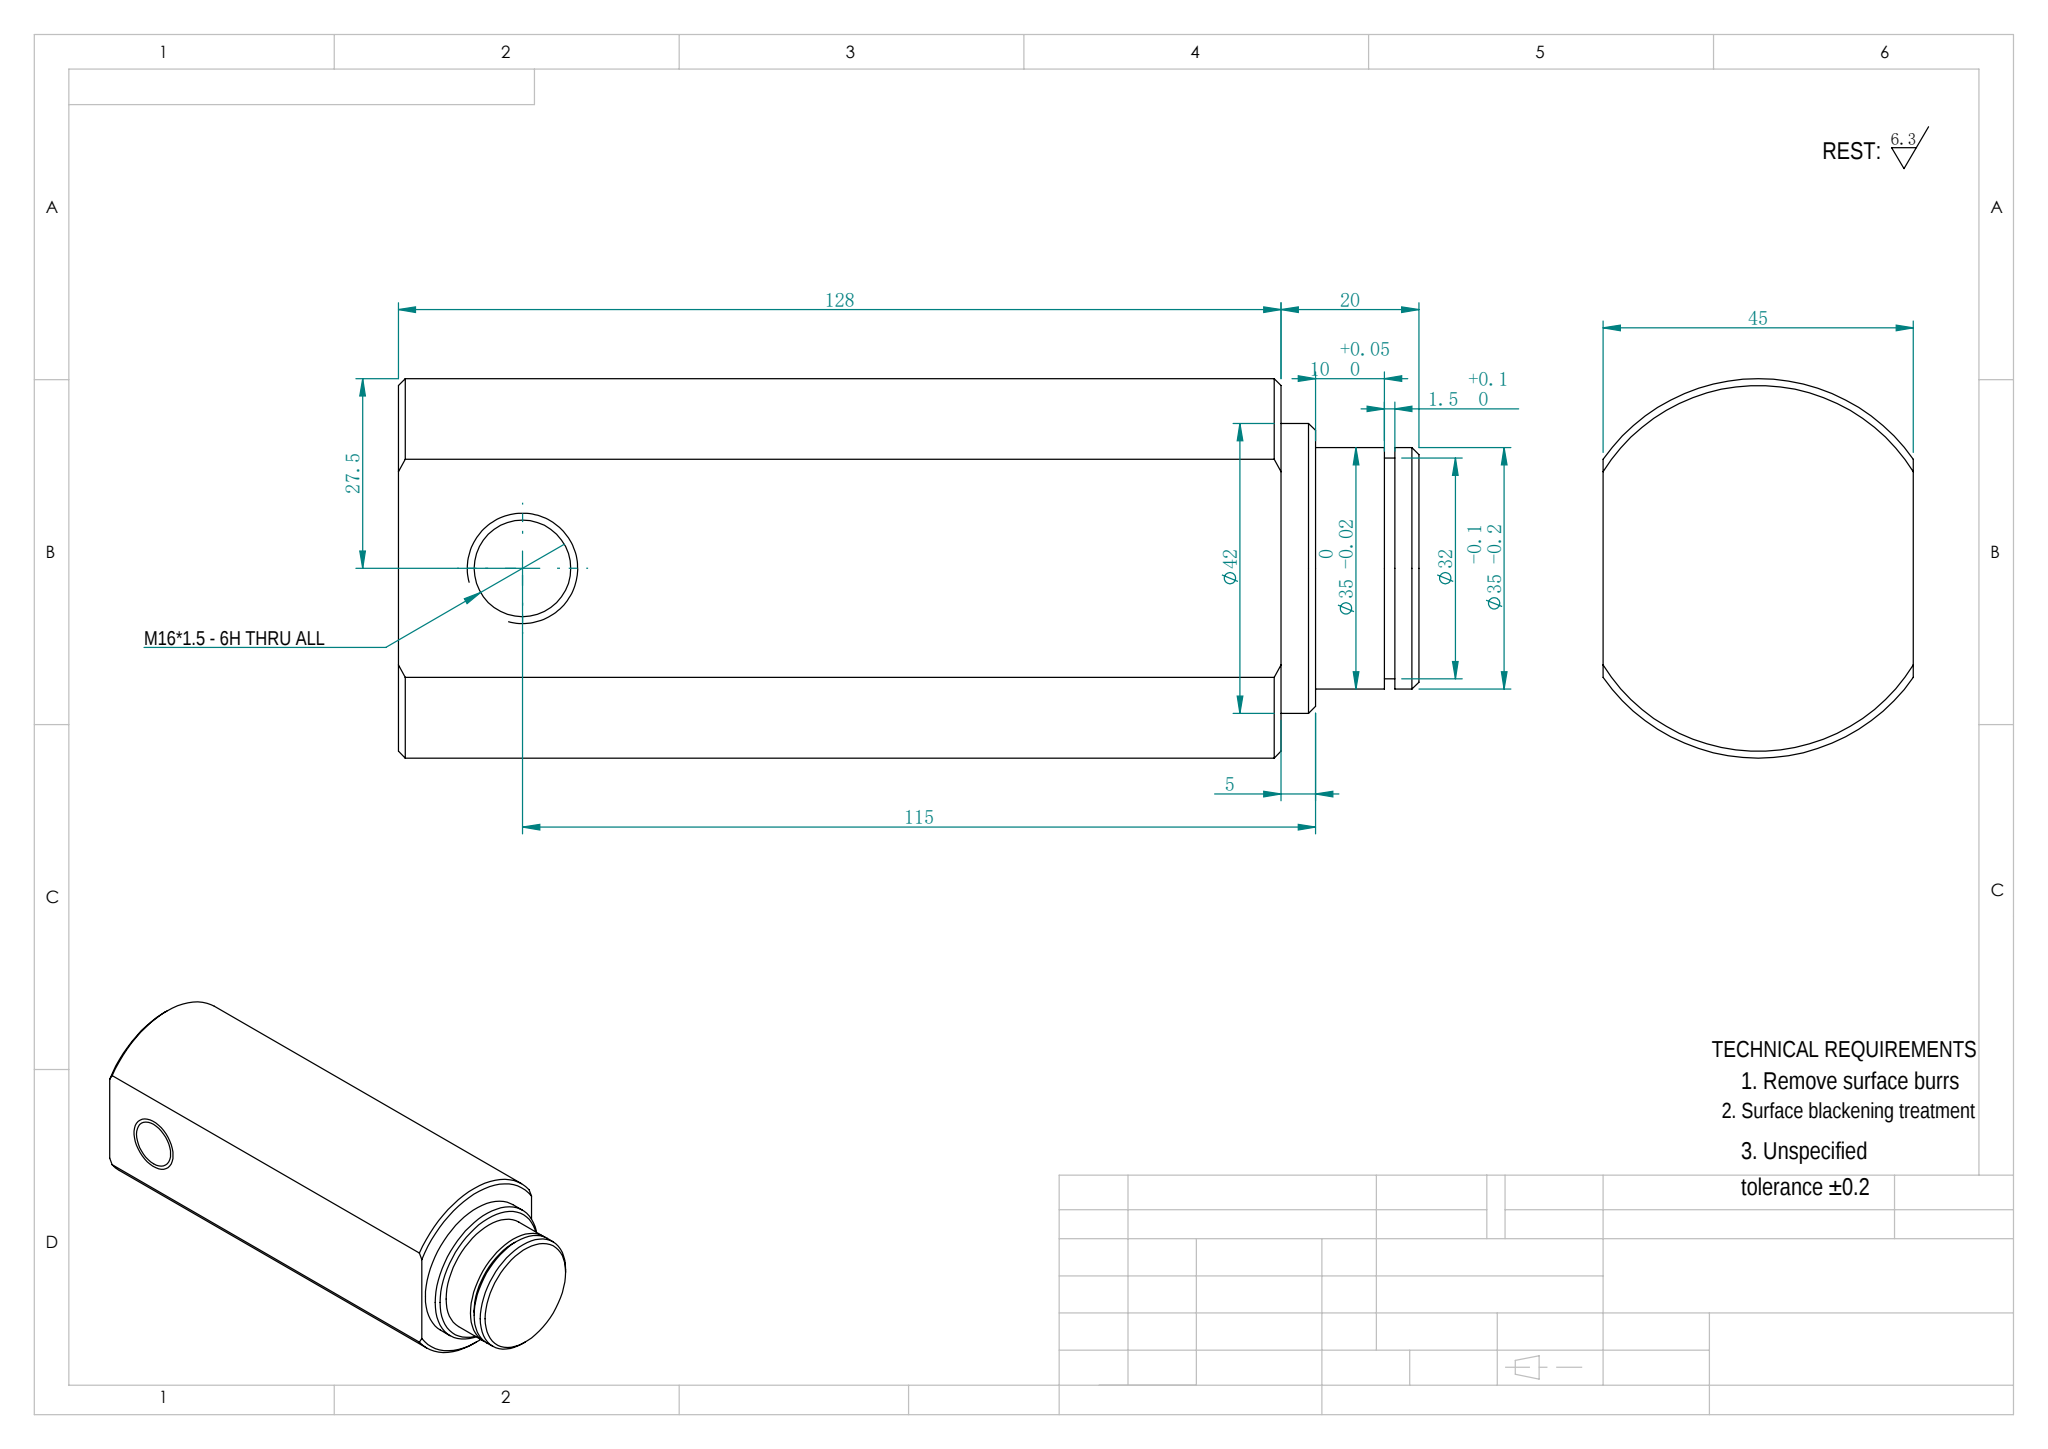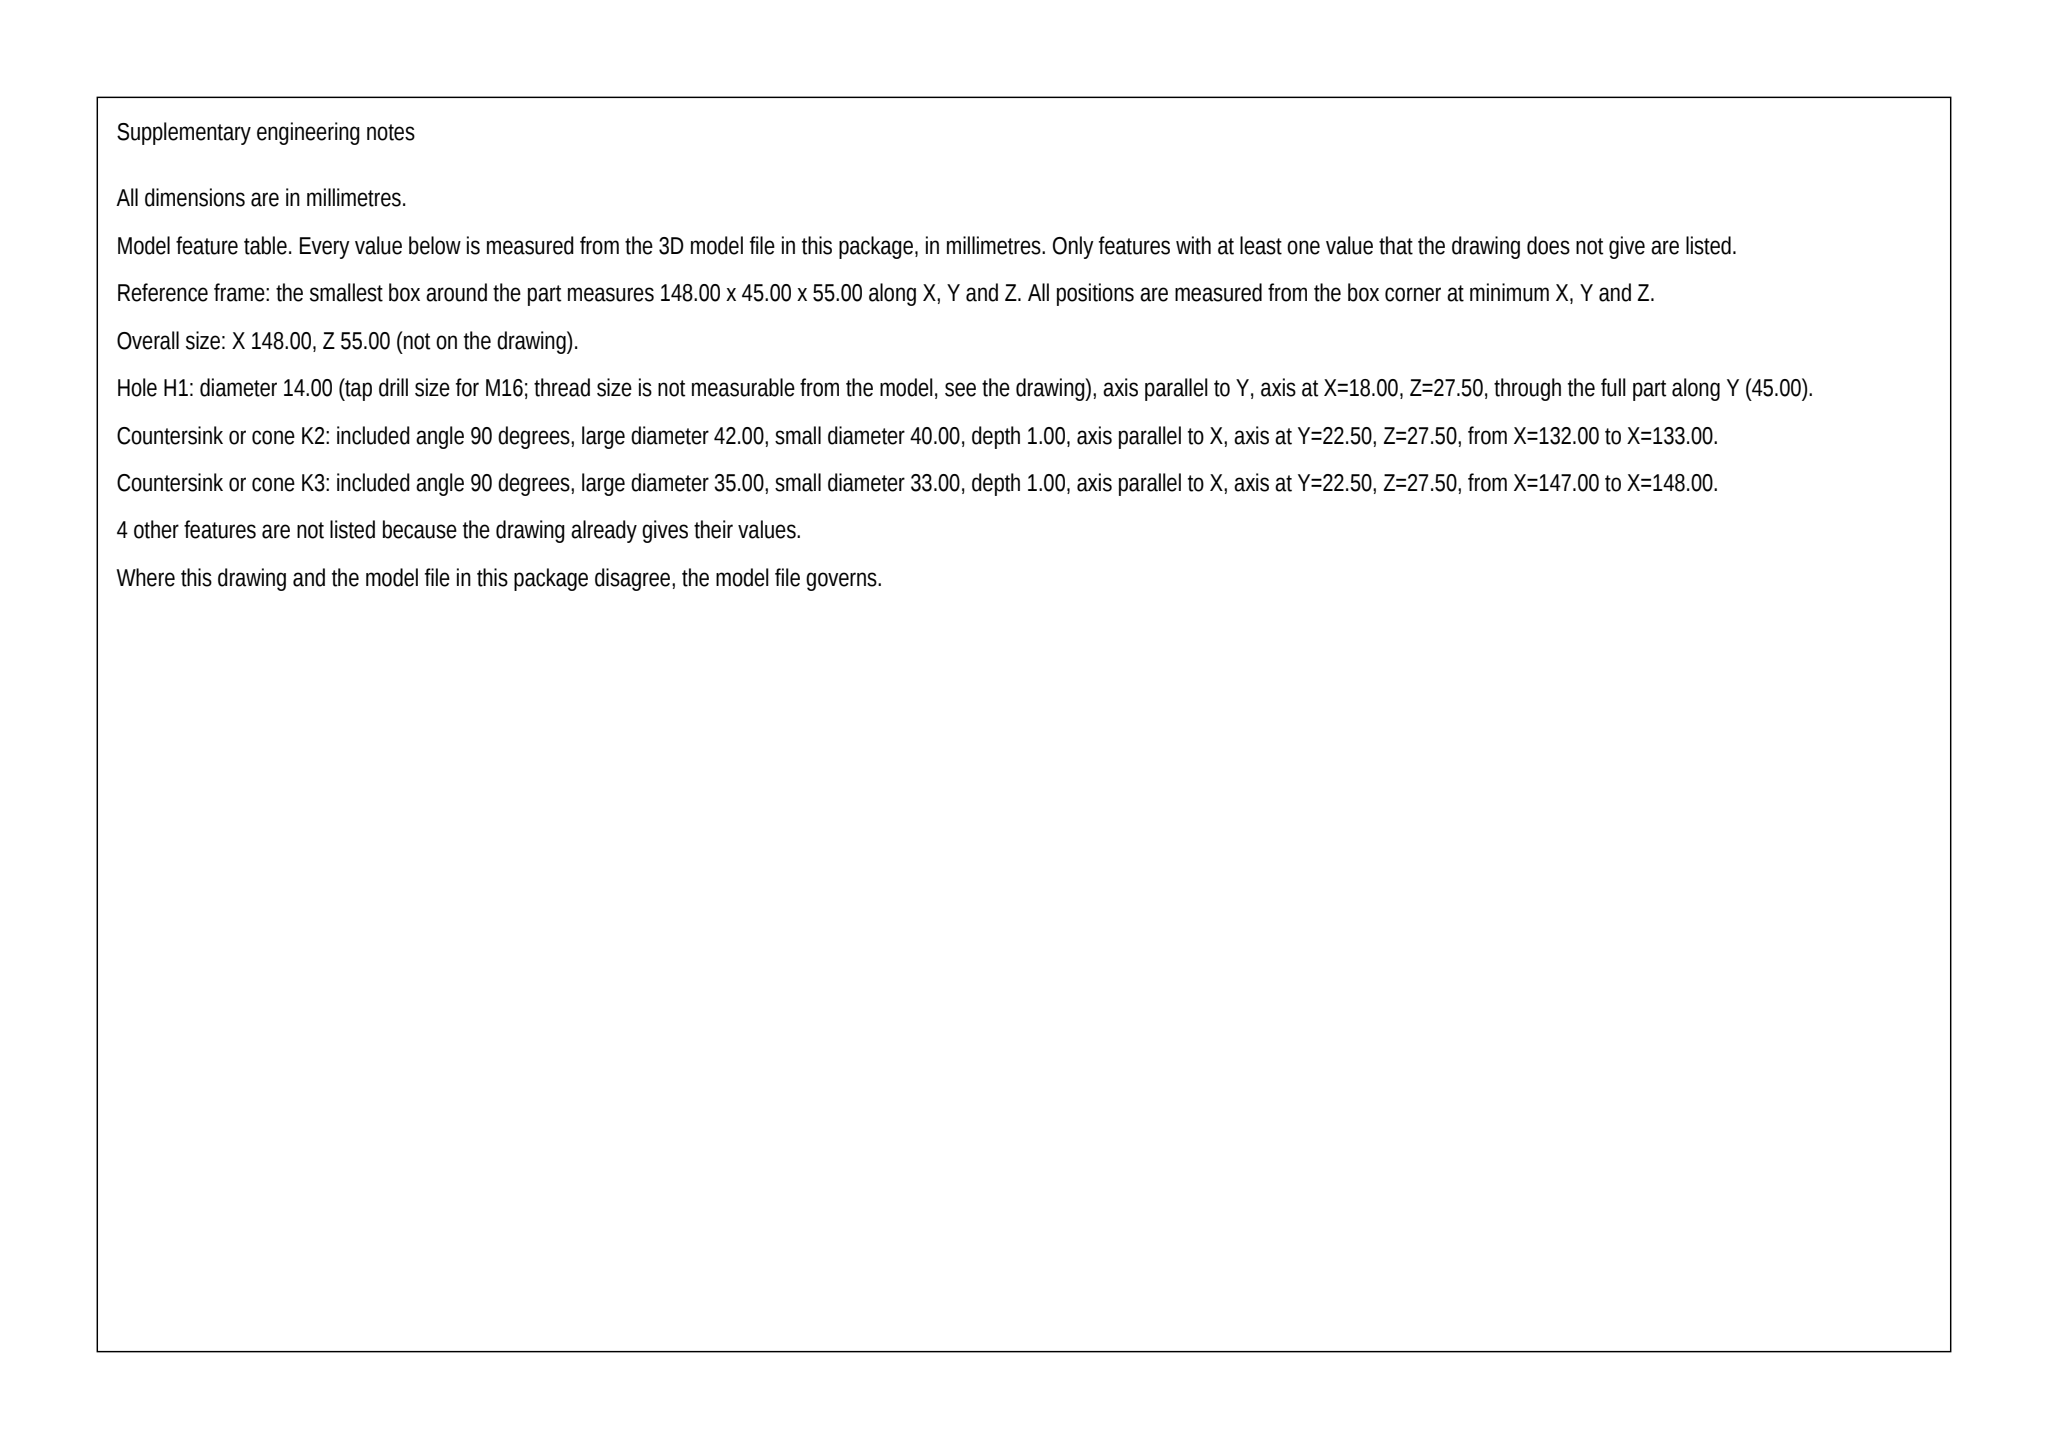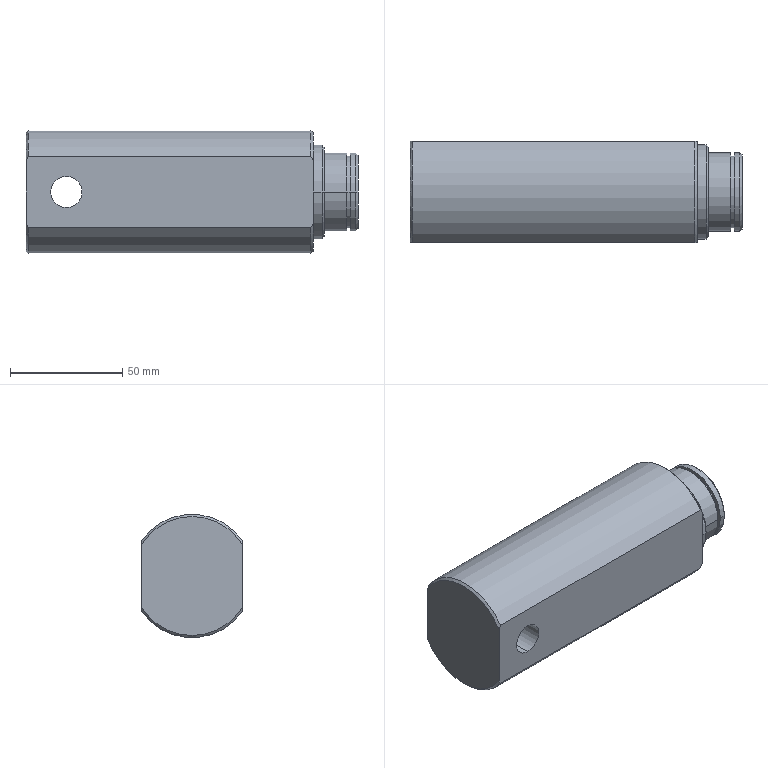Part | SolidWorks | mm | 1 solid | 28 faces | box 148 x 45 x 55 mm | volume 290559 mm3 | cylinder 12 | cone 8 | plane 8 | commonest cylinder face diameters 35 x4 14 x2 32 x2 42 x2 55 x2
build123d program:
from build123d import *

# Parameters (mm, degrees)
SKETCH2_OUTSIDE_W   = 90.438
SKETCH2_OUTSIDE_H   = 90.438
SKETCH2_OUTSIDE_W_2 = 65
SKETCH2_OUTSIDE_H_2 = 45
CUT_EXTRUDE1_DEPTH  = 154.025
M16_TAPPED_HOLE1_D  = 14
CHAMFER1_SIZE       = 1


with BuildPart() as part:
    # Sketch1 → Revolve1 (revolve)
    with BuildSketch(Plane.XY):
        Polygon((0, 0), (0, 27.5), (128, 27.5), (128, 21), (133, 21), (133, 17.5), (143, 17.5), (143, 16), (144.5, 16), (144.5, 17.5), (148, 17.5), (148, 0), align=None)
    revolve(axis=Axis((148, 0, 0), (-1, 0, 0)))

    # Sketch2 outside → Cut-Extrude1 (cut, through all)
    with BuildSketch(Plane.ZY):
        Rectangle(SKETCH2_OUTSIDE_W, SKETCH2_OUTSIDE_H)
        Rectangle(SKETCH2_OUTSIDE_W_2, SKETCH2_OUTSIDE_H_2, mode=Mode.SUBTRACT)
    extrude(amount=-CUT_EXTRUDE1_DEPTH, mode=Mode.SUBTRACT)

    # M16 Tapped Hole1 (through all)
    with Locations(Plane(origin=(0, 22.5, 0), x_dir=(1, 0, 0), z_dir=(0, 1, 0))):
        with Locations((18, 0)):
            Hole(M16_TAPPED_HOLE1_D / 2)

    # Chamfer1
    chamfer1_edges = [part.edges().sort_by_distance(p)[0] for p in [
        (133, -21, 0),
        (128, 0, 27.5),
        (0, 0, 27.5),
        (128, 0, -27.5),
        (0, 0, -27.5),
        (148, -17.5, 0),
    ]]
    chamfer(chamfer1_edges, length=CHAMFER1_SIZE)


solid = part.part
STEP:
#1=CARTESIAN_POINT('',(133.,20.,0.));
#2=VERTEX_POINT('',#1);
#3=CARTESIAN_POINT('',(133.,-20.,0.));
#4=VERTEX_POINT('',#3);
#5=CARTESIAN_POINT('',(133.,0.,0.));
#6=DIRECTION('',(1.,0.,0.));
#7=DIRECTION('',(0.,1.,0.));
#8=AXIS2_PLACEMENT_3D('',#5,#6,#7);
#9=CIRCLE('',#8,20.);
#10=EDGE_CURVE('',#2,#4,#9,.T.);
#11=ORIENTED_EDGE('',*,*,#10,.F.);
#12=CARTESIAN_POINT('',(132.,21.,0.));
#13=VERTEX_POINT('',#12);
#14=CARTESIAN_POINT('',(133.,20.,0.));
#15=DIRECTION('',(-0.7071,0.7071,0.));
#16=VECTOR('',#15,1000.);
#17=LINE('',#14,#16);
#18=EDGE_CURVE('',#2,#13,#17,.T.);
#19=ORIENTED_EDGE('',*,*,#18,.T.);
#20=CARTESIAN_POINT('',(132.,-21.,0.));
#21=VERTEX_POINT('',#20);
#22=CARTESIAN_POINT('',(132.,0.,0.));
#23=DIRECTION('',(-1.,-0.,0.));
#24=DIRECTION('',(0.,1.,0.));
#25=AXIS2_PLACEMENT_3D('',#22,#23,#24);
#26=CIRCLE('',#25,21.);
#27=EDGE_CURVE('',#21,#13,#26,.T.);
#28=ORIENTED_EDGE('',*,*,#27,.F.);
#29=CARTESIAN_POINT('',(133.,-20.,0.));
#30=DIRECTION('',(-0.7071,-0.7071,0.));
#31=VECTOR('',#30,1000.);
#32=LINE('',#29,#31);
#33=EDGE_CURVE('',#4,#21,#32,.T.);
#34=ORIENTED_EDGE('',*,*,#33,.F.);
#35=EDGE_LOOP('',(#11,#19,#28,#34));
#36=FACE_OUTER_BOUND('',#35,.T.);
#37=CARTESIAN_POINT('',(133.,0.,0.));
#38=DIRECTION('',(-1.,-0.,0.));
#39=DIRECTION('',(0.,-1.,0.));
#40=AXIS2_PLACEMENT_3D('',#37,#38,#39);
#41=CONICAL_SURFACE('',#40,20.,0.7854);
#42=ADVANCED_FACE('',(#36),#41,.T.);
#43=CARTESIAN_POINT('',(148.,16.5,0.));
#44=VERTEX_POINT('',#43);
#45=CARTESIAN_POINT('',(148.,-16.5,0.));
#46=VERTEX_POINT('',#45);
#47=CARTESIAN_POINT('',(148.,0.,0.));
#48=DIRECTION('',(1.,0.,0.));
#49=DIRECTION('',(0.,1.,0.));
#50=AXIS2_PLACEMENT_3D('',#47,#48,#49);
#51=CIRCLE('',#50,16.5);
#52=EDGE_CURVE('',#44,#46,#51,.T.);
#53=ORIENTED_EDGE('',*,*,#52,.F.);
#54=CARTESIAN_POINT('',(147.,17.5,0.));
#55=VERTEX_POINT('',#54);
#56=CARTESIAN_POINT('',(148.,16.5,0.));
#57=DIRECTION('',(-0.7071,0.7071,0.));
#58=VECTOR('',#57,1000.);
#59=LINE('',#56,#58);
#60=EDGE_CURVE('',#44,#55,#59,.T.);
#61=ORIENTED_EDGE('',*,*,#60,.T.);
#62=CARTESIAN_POINT('',(147.,-17.5,0.));
#63=VERTEX_POINT('',#62);
#64=CARTESIAN_POINT('',(147.,0.,0.));
#65=DIRECTION('',(-1.,-0.,0.));
#66=DIRECTION('',(0.,1.,0.));
#67=AXIS2_PLACEMENT_3D('',#64,#65,#66);
#68=CIRCLE('',#67,17.5);
#69=EDGE_CURVE('',#63,#55,#68,.T.);
#70=ORIENTED_EDGE('',*,*,#69,.F.);
#71=CARTESIAN_POINT('',(148.,-16.5,0.));
#72=DIRECTION('',(-0.7071,-0.7071,0.));
#73=VECTOR('',#72,1000.);
#74=LINE('',#71,#73);
#75=EDGE_CURVE('',#46,#63,#74,.T.);
#76=ORIENTED_EDGE('',*,*,#75,.F.);
#77=EDGE_LOOP('',(#53,#61,#70,#76));
#78=FACE_OUTER_BOUND('',#77,.T.);
#79=CARTESIAN_POINT('',(148.,0.,0.));
#80=DIRECTION('',(-1.,-0.,0.));
#81=DIRECTION('',(0.,-1.,0.));
#82=AXIS2_PLACEMENT_3D('',#79,#80,#81);
#83=CONICAL_SURFACE('',#82,16.5,0.7854);
#84=ADVANCED_FACE('',(#78),#83,.T.);
#85=CARTESIAN_POINT('',(18.,-22.5,-7.));
#86=VERTEX_POINT('',#85);
#87=CARTESIAN_POINT('',(18.,-22.5,7.));
#88=VERTEX_POINT('',#87);
#89=CARTESIAN_POINT('',(18.,-22.5,0.));
#90=DIRECTION('',(0.,1.,0.));
#91=DIRECTION('',(0.,0.,1.));
#92=AXIS2_PLACEMENT_3D('',#89,#90,#91);
#93=CIRCLE('',#92,7.);
#94=EDGE_CURVE('',#86,#88,#93,.T.);
#95=ORIENTED_EDGE('',*,*,#94,.F.);
#96=CARTESIAN_POINT('',(18.,22.5,-7.));
#97=VERTEX_POINT('',#96);
#98=CARTESIAN_POINT('',(18.,22.5,-7.));
#99=DIRECTION('',(0.,1.,0.));
#100=VECTOR('',#99,1000.);
#101=LINE('',#98,#100);
#102=EDGE_CURVE('',#86,#97,#101,.T.);
#103=ORIENTED_EDGE('',*,*,#102,.T.);
#104=CARTESIAN_POINT('',(18.,22.5,7.));
#105=VERTEX_POINT('',#104);
#106=CARTESIAN_POINT('',(18.,22.5,0.));
#107=DIRECTION('',(0.,1.,0.));
#108=DIRECTION('',(0.,0.,1.));
#109=AXIS2_PLACEMENT_3D('',#106,#107,#108);
#110=CIRCLE('',#109,7.);
#111=EDGE_CURVE('',#97,#105,#110,.T.);
#112=ORIENTED_EDGE('',*,*,#111,.T.);
#113=CARTESIAN_POINT('',(18.,22.5,7.));
#114=DIRECTION('',(0.,1.,0.));
#115=VECTOR('',#114,1000.);
#116=LINE('',#113,#115);
#117=EDGE_CURVE('',#88,#105,#116,.T.);
#118=ORIENTED_EDGE('',*,*,#117,.F.);
#119=EDGE_LOOP('',(#95,#103,#112,#118));
#120=FACE_OUTER_BOUND('',#119,.T.);
#121=CARTESIAN_POINT('',(18.,22.5,0.));
#122=DIRECTION('',(0.,1.,0.));
#123=DIRECTION('',(0.,0.,1.));
#124=AXIS2_PLACEMENT_3D('',#121,#122,#123);
#125=CYLINDRICAL_SURFACE('',#124,7.);
#126=ADVANCED_FACE('',(#120),#125,.F.);
#127=CARTESIAN_POINT('',(144.5,17.5,0.));
#128=VERTEX_POINT('',#127);
#129=CARTESIAN_POINT('',(144.5,-17.5,0.));
#130=VERTEX_POINT('',#129);
#131=CARTESIAN_POINT('',(144.5,0.,0.));
#132=DIRECTION('',(1.,0.,0.));
#133=DIRECTION('',(0.,1.,0.));
#134=AXIS2_PLACEMENT_3D('',#131,#132,#133);
#135=CIRCLE('',#134,17.5);
#136=EDGE_CURVE('',#128,#130,#135,.T.);
#137=ORIENTED_EDGE('',*,*,#136,.T.);
#138=CARTESIAN_POINT('',(148.,-17.5,0.));
#139=DIRECTION('',(1.,0.,0.));
#140=VECTOR('',#139,1000.);
#141=LINE('',#138,#140);
#142=EDGE_CURVE('',#130,#63,#141,.T.);
#143=ORIENTED_EDGE('',*,*,#142,.T.);
#144=ORIENTED_EDGE('',*,*,#69,.T.);
#145=CARTESIAN_POINT('',(148.,17.5,0.));
#146=DIRECTION('',(1.,0.,0.));
#147=VECTOR('',#146,1000.);
#148=LINE('',#145,#147);
#149=EDGE_CURVE('',#128,#55,#148,.T.);
#150=ORIENTED_EDGE('',*,*,#149,.F.);
#151=EDGE_LOOP('',(#137,#143,#144,#150));
#152=FACE_OUTER_BOUND('',#151,.T.);
#153=CARTESIAN_POINT('',(148.,0.,0.));
#154=DIRECTION('',(1.,0.,0.));
#155=DIRECTION('',(0.,1.,0.));
#156=AXIS2_PLACEMENT_3D('',#153,#154,#155);
#157=CYLINDRICAL_SURFACE('',#156,17.5);
#158=ADVANCED_FACE('',(#152),#157,.T.);
#159=CARTESIAN_POINT('',(143.,16.,0.));
#160=VERTEX_POINT('',#159);
#161=CARTESIAN_POINT('',(143.,-16.,0.));
#162=VERTEX_POINT('',#161);
#163=CARTESIAN_POINT('',(143.,0.,0.));
#164=DIRECTION('',(1.,0.,0.));
#165=DIRECTION('',(0.,1.,0.));
#166=AXIS2_PLACEMENT_3D('',#163,#164,#165);
#167=CIRCLE('',#166,16.);
#168=EDGE_CURVE('',#160,#162,#167,.T.);
#169=ORIENTED_EDGE('',*,*,#168,.T.);
#170=CARTESIAN_POINT('',(144.5,-16.,0.));
#171=VERTEX_POINT('',#170);
#172=CARTESIAN_POINT('',(148.,-16.,0.));
#173=DIRECTION('',(1.,0.,0.));
#174=VECTOR('',#173,1000.);
#175=LINE('',#172,#174);
#176=EDGE_CURVE('',#162,#171,#175,.T.);
#177=ORIENTED_EDGE('',*,*,#176,.T.);
#178=CARTESIAN_POINT('',(144.5,16.,0.));
#179=VERTEX_POINT('',#178);
#180=CARTESIAN_POINT('',(144.5,0.,0.));
#181=DIRECTION('',(1.,0.,0.));
#182=DIRECTION('',(0.,1.,0.));
#183=AXIS2_PLACEMENT_3D('',#180,#181,#182);
#184=CIRCLE('',#183,16.);
#185=EDGE_CURVE('',#179,#171,#184,.T.);
#186=ORIENTED_EDGE('',*,*,#185,.F.);
#187=CARTESIAN_POINT('',(148.,16.,0.));
#188=DIRECTION('',(1.,0.,0.));
#189=VECTOR('',#188,1000.);
#190=LINE('',#187,#189);
#191=EDGE_CURVE('',#160,#179,#190,.T.);
#192=ORIENTED_EDGE('',*,*,#191,.F.);
#193=EDGE_LOOP('',(#169,#177,#186,#192));
#194=FACE_OUTER_BOUND('',#193,.T.);
#195=CARTESIAN_POINT('',(148.,0.,0.));
#196=DIRECTION('',(1.,0.,0.));
#197=DIRECTION('',(0.,1.,0.));
#198=AXIS2_PLACEMENT_3D('',#195,#196,#197);
#199=CYLINDRICAL_SURFACE('',#198,16.);
#200=ADVANCED_FACE('',(#194),#199,.T.);
#201=CARTESIAN_POINT('',(133.,17.5,0.));
#202=VERTEX_POINT('',#201);
#203=CARTESIAN_POINT('',(133.,-17.5,0.));
#204=VERTEX_POINT('',#203);
#205=CARTESIAN_POINT('',(133.,0.,0.));
#206=DIRECTION('',(1.,0.,0.));
#207=DIRECTION('',(0.,1.,0.));
#208=AXIS2_PLACEMENT_3D('',#205,#206,#207);
#209=CIRCLE('',#208,17.5);
#210=EDGE_CURVE('',#202,#204,#209,.T.);
#211=ORIENTED_EDGE('',*,*,#210,.T.);
#212=CARTESIAN_POINT('',(143.,-17.5,0.));
#213=VERTEX_POINT('',#212);
#214=CARTESIAN_POINT('',(148.,-17.5,0.));
#215=DIRECTION('',(1.,0.,0.));
#216=VECTOR('',#215,1000.);
#217=LINE('',#214,#216);
#218=EDGE_CURVE('',#204,#213,#217,.T.);
#219=ORIENTED_EDGE('',*,*,#218,.T.);
#220=CARTESIAN_POINT('',(143.,17.5,0.));
#221=VERTEX_POINT('',#220);
#222=CARTESIAN_POINT('',(143.,0.,0.));
#223=DIRECTION('',(1.,0.,0.));
#224=DIRECTION('',(0.,1.,0.));
#225=AXIS2_PLACEMENT_3D('',#222,#223,#224);
#226=CIRCLE('',#225,17.5);
#227=EDGE_CURVE('',#221,#213,#226,.T.);
#228=ORIENTED_EDGE('',*,*,#227,.F.);
#229=CARTESIAN_POINT('',(148.,17.5,0.));
#230=DIRECTION('',(1.,0.,0.));
#231=VECTOR('',#230,1000.);
#232=LINE('',#229,#231);
#233=EDGE_CURVE('',#202,#221,#232,.T.);
#234=ORIENTED_EDGE('',*,*,#233,.F.);
#235=EDGE_LOOP('',(#211,#219,#228,#234));
#236=FACE_OUTER_BOUND('',#235,.T.);
#237=CARTESIAN_POINT('',(148.,0.,0.));
#238=DIRECTION('',(1.,0.,0.));
#239=DIRECTION('',(0.,1.,0.));
#240=AXIS2_PLACEMENT_3D('',#237,#238,#239);
#241=CYLINDRICAL_SURFACE('',#240,17.5);
#242=ADVANCED_FACE('',(#236),#241,.T.);
#243=CARTESIAN_POINT('',(128.,21.,0.));
#244=VERTEX_POINT('',#243);
#245=CARTESIAN_POINT('',(128.,-21.,0.));
#246=VERTEX_POINT('',#245);
#247=CARTESIAN_POINT('',(128.,0.,0.));
#248=DIRECTION('',(1.,0.,0.));
#249=DIRECTION('',(0.,1.,0.));
#250=AXIS2_PLACEMENT_3D('',#247,#248,#249);
#251=CIRCLE('',#250,21.);
#252=EDGE_CURVE('',#244,#246,#251,.T.);
#253=ORIENTED_EDGE('',*,*,#252,.T.);
#254=CARTESIAN_POINT('',(148.,-21.,0.));
#255=DIRECTION('',(1.,0.,0.));
#256=VECTOR('',#255,1000.);
#257=LINE('',#254,#256);
#258=EDGE_CURVE('',#246,#21,#257,.T.);
#259=ORIENTED_EDGE('',*,*,#258,.T.);
#260=ORIENTED_EDGE('',*,*,#27,.T.);
#261=CARTESIAN_POINT('',(148.,21.,0.));
#262=DIRECTION('',(1.,0.,0.));
#263=VECTOR('',#262,1000.);
#264=LINE('',#261,#263);
#265=EDGE_CURVE('',#244,#13,#264,.T.);
#266=ORIENTED_EDGE('',*,*,#265,.F.);
#267=EDGE_LOOP('',(#253,#259,#260,#266));
#268=FACE_OUTER_BOUND('',#267,.T.);
#269=CARTESIAN_POINT('',(148.,0.,0.));
#270=DIRECTION('',(1.,0.,0.));
#271=DIRECTION('',(0.,1.,0.));
#272=AXIS2_PLACEMENT_3D('',#269,#270,#271);
#273=CYLINDRICAL_SURFACE('',#272,21.);
#274=ADVANCED_FACE('',(#268),#273,.T.);
#275=CARTESIAN_POINT('',(0.,-22.5,-14.));
#276=VERTEX_POINT('',#275);
#277=CARTESIAN_POINT('',(0.,-22.5,14.));
#278=VERTEX_POINT('',#277);
#279=CARTESIAN_POINT('',(0.,-22.5,-32.5));
#280=DIRECTION('',(0.,0.,1.));
#281=VECTOR('',#280,1000.);
#282=LINE('',#279,#281);
#283=EDGE_CURVE('',#276,#278,#282,.T.);
#284=ORIENTED_EDGE('',*,*,#283,.T.);
#285=CARTESIAN_POINT('',(-0.,22.5,14.));
#286=VERTEX_POINT('',#285);
#287=CARTESIAN_POINT('',(0.,0.,0.));
#288=DIRECTION('',(-1.,-0.,0.));
#289=DIRECTION('',(0.,-1.,0.));
#290=AXIS2_PLACEMENT_3D('',#287,#288,#289);
#291=CIRCLE('',#290,26.5);
#292=EDGE_CURVE('',#278,#286,#291,.T.);
#293=ORIENTED_EDGE('',*,*,#292,.T.);
#294=CARTESIAN_POINT('',(-0.,22.5,-14.));
#295=VERTEX_POINT('',#294);
#296=CARTESIAN_POINT('',(-0.,22.5,-32.5));
#297=DIRECTION('',(0.,0.,-1.));
#298=VECTOR('',#297,1000.);
#299=LINE('',#296,#298);
#300=EDGE_CURVE('',#286,#295,#299,.T.);
#301=ORIENTED_EDGE('',*,*,#300,.T.);
#302=CARTESIAN_POINT('',(0.,0.,0.));
#303=DIRECTION('',(-1.,-0.,0.));
#304=DIRECTION('',(0.,-1.,0.));
#305=AXIS2_PLACEMENT_3D('',#302,#303,#304);
#306=CIRCLE('',#305,26.5);
#307=EDGE_CURVE('',#295,#276,#306,.T.);
#308=ORIENTED_EDGE('',*,*,#307,.T.);
#309=EDGE_LOOP('',(#284,#293,#301,#308));
#310=FACE_OUTER_BOUND('',#309,.T.);
#311=CARTESIAN_POINT('',(0.,0.,0.));
#312=DIRECTION('',(-1.,-0.,0.));
#313=DIRECTION('',(0.,-1.,0.));
#314=AXIS2_PLACEMENT_3D('',#311,#312,#313);
#315=PLANE('',#314);
#316=ADVANCED_FACE('',(#310),#315,.T.);
#317=CARTESIAN_POINT('',(127.,-22.5,-15.811));
#318=VERTEX_POINT('',#317);
#319=CARTESIAN_POINT('',(1.,-22.5,-15.811));
#320=VERTEX_POINT('',#319);
#321=CARTESIAN_POINT('',(148.,-22.5,-15.811));
#322=DIRECTION('',(-1.,-0.,0.));
#323=VECTOR('',#322,1000.);
#324=LINE('',#321,#323);
#325=EDGE_CURVE('',#318,#320,#324,.T.);
#326=ORIENTED_EDGE('',*,*,#325,.T.);
#327=CARTESIAN_POINT('',(1.,22.5,-15.811));
#328=VERTEX_POINT('',#327);
#329=CARTESIAN_POINT('',(1.,0.,0.));
#330=DIRECTION('',(1.,0.,0.));
#331=DIRECTION('',(0.,-1.,0.));
#332=AXIS2_PLACEMENT_3D('',#329,#330,#331);
#333=CIRCLE('',#332,27.5);
#334=EDGE_CURVE('',#320,#328,#333,.T.);
#335=ORIENTED_EDGE('',*,*,#334,.T.);
#336=CARTESIAN_POINT('',(127.,22.5,-15.811));
#337=VERTEX_POINT('',#336);
#338=CARTESIAN_POINT('',(148.,22.5,-15.811));
#339=DIRECTION('',(1.,0.,0.));
#340=VECTOR('',#339,1000.);
#341=LINE('',#338,#340);
#342=EDGE_CURVE('',#328,#337,#341,.T.);
#343=ORIENTED_EDGE('',*,*,#342,.T.);
#344=CARTESIAN_POINT('',(127.,0.,0.));
#345=DIRECTION('',(-1.,-0.,0.));
#346=DIRECTION('',(0.,1.,0.));
#347=AXIS2_PLACEMENT_3D('',#344,#345,#346);
#348=CIRCLE('',#347,27.5);
#349=EDGE_CURVE('',#337,#318,#348,.T.);
#350=ORIENTED_EDGE('',*,*,#349,.T.);
#351=EDGE_LOOP('',(#326,#335,#343,#350));
#352=FACE_OUTER_BOUND('',#351,.T.);
#353=CARTESIAN_POINT('',(148.,0.,0.));
#354=DIRECTION('',(1.,0.,0.));
#355=DIRECTION('',(0.,1.,0.));
#356=AXIS2_PLACEMENT_3D('',#353,#354,#355);
#357=CYLINDRICAL_SURFACE('',#356,27.5);
#358=ADVANCED_FACE('',(#352),#357,.T.);
#359=CARTESIAN_POINT('',(127.,22.5,15.811));
#360=VERTEX_POINT('',#359);
#361=CARTESIAN_POINT('',(1.,22.5,15.811));
#362=VERTEX_POINT('',#361);
#363=CARTESIAN_POINT('',(148.,22.5,15.811));
#364=DIRECTION('',(-1.,-0.,0.));
#365=VECTOR('',#364,1000.);
#366=LINE('',#363,#365);
#367=EDGE_CURVE('',#360,#362,#366,.T.);
#368=ORIENTED_EDGE('',*,*,#367,.T.);
#369=CARTESIAN_POINT('',(1.,-22.5,15.811));
#370=VERTEX_POINT('',#369);
#371=CARTESIAN_POINT('',(1.,0.,0.));
#372=DIRECTION('',(1.,0.,0.));
#373=DIRECTION('',(0.,-1.,0.));
#374=AXIS2_PLACEMENT_3D('',#371,#372,#373);
#375=CIRCLE('',#374,27.5);
#376=EDGE_CURVE('',#362,#370,#375,.T.);
#377=ORIENTED_EDGE('',*,*,#376,.T.);
#378=CARTESIAN_POINT('',(127.,-22.5,15.811));
#379=VERTEX_POINT('',#378);
#380=CARTESIAN_POINT('',(148.,-22.5,15.811));
#381=DIRECTION('',(1.,0.,0.));
#382=VECTOR('',#381,1000.);
#383=LINE('',#380,#382);
#384=EDGE_CURVE('',#370,#379,#383,.T.);
#385=ORIENTED_EDGE('',*,*,#384,.T.);
#386=CARTESIAN_POINT('',(127.,0.,0.));
#387=DIRECTION('',(-1.,-0.,0.));
#388=DIRECTION('',(0.,1.,0.));
#389=AXIS2_PLACEMENT_3D('',#386,#387,#388);
#390=CIRCLE('',#389,27.5);
#391=EDGE_CURVE('',#379,#360,#390,.T.);
#392=ORIENTED_EDGE('',*,*,#391,.T.);
#393=EDGE_LOOP('',(#368,#377,#385,#392));
#394=FACE_OUTER_BOUND('',#393,.T.);
#395=CARTESIAN_POINT('',(148.,0.,0.));
#396=DIRECTION('',(1.,0.,0.));
#397=DIRECTION('',(0.,1.,0.));
#398=AXIS2_PLACEMENT_3D('',#395,#396,#397);
#399=CYLINDRICAL_SURFACE('',#398,27.5);
#400=ADVANCED_FACE('',(#394),#399,.T.);
#401=ORIENTED_EDGE('',*,*,#252,.F.);
#402=CARTESIAN_POINT('',(128.,0.,0.));
#403=DIRECTION('',(1.,0.,0.));
#404=DIRECTION('',(0.,1.,0.));
#405=AXIS2_PLACEMENT_3D('',#402,#403,#404);
#406=CIRCLE('',#405,21.);
#407=EDGE_CURVE('',#246,#244,#406,.T.);
#408=ORIENTED_EDGE('',*,*,#407,.F.);
#409=EDGE_LOOP('',(#401,#408));
#410=FACE_BOUND('',#409,.T.);
#411=CARTESIAN_POINT('',(128.,22.5,-14.));
#412=VERTEX_POINT('',#411);
#413=CARTESIAN_POINT('',(128.,22.5,14.));
#414=VERTEX_POINT('',#413);
#415=CARTESIAN_POINT('',(128.,22.5,0.));
#416=DIRECTION('',(0.,0.,1.));
#417=VECTOR('',#416,1000.);
#418=LINE('',#415,#417);
#419=EDGE_CURVE('',#412,#414,#418,.T.);
#420=ORIENTED_EDGE('',*,*,#419,.T.);
#421=CARTESIAN_POINT('',(128.,-22.5,14.));
#422=VERTEX_POINT('',#421);
#423=CARTESIAN_POINT('',(128.,0.,0.));
#424=DIRECTION('',(1.,0.,0.));
#425=DIRECTION('',(0.,1.,0.));
#426=AXIS2_PLACEMENT_3D('',#423,#424,#425);
#427=CIRCLE('',#426,26.5);
#428=EDGE_CURVE('',#414,#422,#427,.T.);
#429=ORIENTED_EDGE('',*,*,#428,.T.);
#430=CARTESIAN_POINT('',(128.,-22.5,-14.));
#431=VERTEX_POINT('',#430);
#432=CARTESIAN_POINT('',(128.,-22.5,0.));
#433=DIRECTION('',(0.,0.,-1.));
#434=VECTOR('',#433,1000.);
#435=LINE('',#432,#434);
#436=EDGE_CURVE('',#422,#431,#435,.T.);
#437=ORIENTED_EDGE('',*,*,#436,.T.);
#438=CARTESIAN_POINT('',(128.,0.,0.));
#439=DIRECTION('',(1.,0.,0.));
#440=DIRECTION('',(0.,1.,0.));
#441=AXIS2_PLACEMENT_3D('',#438,#439,#440);
#442=CIRCLE('',#441,26.5);
#443=EDGE_CURVE('',#431,#412,#442,.T.);
#444=ORIENTED_EDGE('',*,*,#443,.T.);
#445=EDGE_LOOP('',(#420,#429,#437,#444));
#446=FACE_OUTER_BOUND('',#445,.T.);
#447=CARTESIAN_POINT('',(128.,27.5,0.));
#448=DIRECTION('',(1.,0.,0.));
#449=DIRECTION('',(-0.,1.,0.));
#450=AXIS2_PLACEMENT_3D('',#447,#448,#449);
#451=PLANE('',#450);
#452=ADVANCED_FACE('',(#410,#446),#451,.T.);
#453=ORIENTED_EDGE('',*,*,#258,.F.);
#454=ORIENTED_EDGE('',*,*,#407,.T.);
#455=ORIENTED_EDGE('',*,*,#265,.T.);
#456=CARTESIAN_POINT('',(132.,0.,0.));
#457=DIRECTION('',(-1.,-0.,0.));
#458=DIRECTION('',(0.,1.,0.));
#459=AXIS2_PLACEMENT_3D('',#456,#457,#458);
#460=CIRCLE('',#459,21.);
#461=EDGE_CURVE('',#13,#21,#460,.T.);
#462=ORIENTED_EDGE('',*,*,#461,.T.);
#463=EDGE_LOOP('',(#453,#454,#455,#462));
#464=FACE_OUTER_BOUND('',#463,.T.);
#465=CARTESIAN_POINT('',(148.,0.,0.));
#466=DIRECTION('',(1.,0.,0.));
#467=DIRECTION('',(0.,1.,0.));
#468=AXIS2_PLACEMENT_3D('',#465,#466,#467);
#469=CYLINDRICAL_SURFACE('',#468,21.);
#470=ADVANCED_FACE('',(#464),#469,.T.);
#471=CARTESIAN_POINT('',(133.,0.,0.));
#472=DIRECTION('',(1.,0.,0.));
#473=DIRECTION('',(0.,1.,0.));
#474=AXIS2_PLACEMENT_3D('',#471,#472,#473);
#475=CIRCLE('',#474,20.);
#476=EDGE_CURVE('',#4,#2,#475,.T.);
#477=ORIENTED_EDGE('',*,*,#476,.T.);
#478=ORIENTED_EDGE('',*,*,#10,.T.);
#479=EDGE_LOOP('',(#477,#478));
#480=FACE_OUTER_BOUND('',#479,.T.);
#481=ORIENTED_EDGE('',*,*,#210,.F.);
#482=CARTESIAN_POINT('',(133.,0.,0.));
#483=DIRECTION('',(1.,0.,0.));
#484=DIRECTION('',(0.,1.,0.));
#485=AXIS2_PLACEMENT_3D('',#482,#483,#484);
#486=CIRCLE('',#485,17.5);
#487=EDGE_CURVE('',#204,#202,#486,.T.);
#488=ORIENTED_EDGE('',*,*,#487,.F.);
#489=EDGE_LOOP('',(#481,#488));
#490=FACE_BOUND('',#489,.T.);
#491=CARTESIAN_POINT('',(133.,21.,0.));
#492=DIRECTION('',(1.,0.,0.));
#493=DIRECTION('',(-0.,1.,0.));
#494=AXIS2_PLACEMENT_3D('',#491,#492,#493);
#495=PLANE('',#494);
#496=ADVANCED_FACE('',(#480,#490),#495,.T.);
#497=ORIENTED_EDGE('',*,*,#218,.F.);
#498=ORIENTED_EDGE('',*,*,#487,.T.);
#499=ORIENTED_EDGE('',*,*,#233,.T.);
#500=CARTESIAN_POINT('',(143.,0.,0.));
#501=DIRECTION('',(1.,0.,0.));
#502=DIRECTION('',(0.,1.,0.));
#503=AXIS2_PLACEMENT_3D('',#500,#501,#502);
#504=CIRCLE('',#503,17.5);
#505=EDGE_CURVE('',#213,#221,#504,.T.);
#506=ORIENTED_EDGE('',*,*,#505,.F.);
#507=EDGE_LOOP('',(#497,#498,#499,#506));
#508=FACE_OUTER_BOUND('',#507,.T.);
#509=CARTESIAN_POINT('',(148.,0.,0.));
#510=DIRECTION('',(1.,0.,0.));
#511=DIRECTION('',(0.,1.,0.));
#512=AXIS2_PLACEMENT_3D('',#509,#510,#511);
#513=CYLINDRICAL_SURFACE('',#512,17.5);
#514=ADVANCED_FACE('',(#508),#513,.T.);
#515=ORIENTED_EDGE('',*,*,#227,.T.);
#516=ORIENTED_EDGE('',*,*,#505,.T.);
#517=EDGE_LOOP('',(#515,#516));
#518=FACE_OUTER_BOUND('',#517,.T.);
#519=ORIENTED_EDGE('',*,*,#168,.F.);
#520=CARTESIAN_POINT('',(143.,0.,0.));
#521=DIRECTION('',(1.,0.,0.));
#522=DIRECTION('',(0.,1.,0.));
#523=AXIS2_PLACEMENT_3D('',#520,#521,#522);
#524=CIRCLE('',#523,16.);
#525=EDGE_CURVE('',#162,#160,#524,.T.);
#526=ORIENTED_EDGE('',*,*,#525,.F.);
#527=EDGE_LOOP('',(#519,#526));
#528=FACE_BOUND('',#527,.T.);
#529=CARTESIAN_POINT('',(143.,17.5,0.));
#530=DIRECTION('',(1.,0.,0.));
#531=DIRECTION('',(-0.,1.,0.));
#532=AXIS2_PLACEMENT_3D('',#529,#530,#531);
#533=PLANE('',#532);
#534=ADVANCED_FACE('',(#518,#528),#533,.T.);
#535=ORIENTED_EDGE('',*,*,#176,.F.);
#536=ORIENTED_EDGE('',*,*,#525,.T.);
#537=ORIENTED_EDGE('',*,*,#191,.T.);
#538=CARTESIAN_POINT('',(144.5,0.,0.));
#539=DIRECTION('',(1.,0.,0.));
#540=DIRECTION('',(0.,1.,0.));
#541=AXIS2_PLACEMENT_3D('',#538,#539,#540);
#542=CIRCLE('',#541,16.);
#543=EDGE_CURVE('',#171,#179,#542,.T.);
#544=ORIENTED_EDGE('',*,*,#543,.F.);
#545=EDGE_LOOP('',(#535,#536,#537,#544));
#546=FACE_OUTER_BOUND('',#545,.T.);
#547=CARTESIAN_POINT('',(148.,0.,0.));
#548=DIRECTION('',(1.,0.,0.));
#549=DIRECTION('',(0.,1.,0.));
#550=AXIS2_PLACEMENT_3D('',#547,#548,#549);
#551=CYLINDRICAL_SURFACE('',#550,16.);
#552=ADVANCED_FACE('',(#546),#551,.T.);
#553=ORIENTED_EDGE('',*,*,#185,.T.);
#554=ORIENTED_EDGE('',*,*,#543,.T.);
#555=EDGE_LOOP('',(#553,#554));
#556=FACE_BOUND('',#555,.T.);
#557=ORIENTED_EDGE('',*,*,#136,.F.);
#558=CARTESIAN_POINT('',(144.5,0.,0.));
#559=DIRECTION('',(1.,0.,0.));
#560=DIRECTION('',(0.,1.,0.));
#561=AXIS2_PLACEMENT_3D('',#558,#559,#560);
#562=CIRCLE('',#561,17.5);
#563=EDGE_CURVE('',#130,#128,#562,.T.);
#564=ORIENTED_EDGE('',*,*,#563,.F.);
#565=EDGE_LOOP('',(#557,#564));
#566=FACE_OUTER_BOUND('',#565,.T.);
#567=CARTESIAN_POINT('',(144.5,17.5,0.));
#568=DIRECTION('',(-1.,-0.,0.));
#569=DIRECTION('',(0.,-1.,0.));
#570=AXIS2_PLACEMENT_3D('',#567,#568,#569);
#571=PLANE('',#570);
#572=ADVANCED_FACE('',(#556,#566),#571,.T.);
#573=ORIENTED_EDGE('',*,*,#142,.F.);
#574=ORIENTED_EDGE('',*,*,#563,.T.);
#575=ORIENTED_EDGE('',*,*,#149,.T.);
#576=CARTESIAN_POINT('',(147.,0.,0.));
#577=DIRECTION('',(-1.,-0.,0.));
#578=DIRECTION('',(0.,1.,0.));
#579=AXIS2_PLACEMENT_3D('',#576,#577,#578);
#580=CIRCLE('',#579,17.5);
#581=EDGE_CURVE('',#55,#63,#580,.T.);
#582=ORIENTED_EDGE('',*,*,#581,.T.);
#583=EDGE_LOOP('',(#573,#574,#575,#582));
#584=FACE_OUTER_BOUND('',#583,.T.);
#585=CARTESIAN_POINT('',(148.,0.,0.));
#586=DIRECTION('',(1.,0.,0.));
#587=DIRECTION('',(0.,1.,0.));
#588=AXIS2_PLACEMENT_3D('',#585,#586,#587);
#589=CYLINDRICAL_SURFACE('',#588,17.5);
#590=ADVANCED_FACE('',(#584),#589,.T.);
#591=CARTESIAN_POINT('',(148.,0.,0.));
#592=DIRECTION('',(1.,0.,0.));
#593=DIRECTION('',(0.,1.,0.));
#594=AXIS2_PLACEMENT_3D('',#591,#592,#593);
#595=CIRCLE('',#594,16.5);
#596=EDGE_CURVE('',#46,#44,#595,.T.);
#597=ORIENTED_EDGE('',*,*,#596,.T.);
#598=ORIENTED_EDGE('',*,*,#52,.T.);
#599=EDGE_LOOP('',(#597,#598));
#600=FACE_OUTER_BOUND('',#599,.T.);
#601=CARTESIAN_POINT('',(148.,17.5,0.));
#602=DIRECTION('',(1.,0.,0.));
#603=DIRECTION('',(-0.,1.,0.));
#604=AXIS2_PLACEMENT_3D('',#601,#602,#603);
#605=PLANE('',#604);
#606=ADVANCED_FACE('',(#600),#605,.T.);
#607=CARTESIAN_POINT('',(18.,22.5,0.));
#608=DIRECTION('',(0.,1.,0.));
#609=DIRECTION('',(0.,0.,1.));
#610=AXIS2_PLACEMENT_3D('',#607,#608,#609);
#611=CIRCLE('',#610,7.);
#612=EDGE_CURVE('',#105,#97,#611,.T.);
#613=ORIENTED_EDGE('',*,*,#612,.F.);
#614=ORIENTED_EDGE('',*,*,#111,.F.);
#615=EDGE_LOOP('',(#613,#614));
#616=FACE_BOUND('',#615,.T.);
#617=ORIENTED_EDGE('',*,*,#300,.F.);
#618=CARTESIAN_POINT('',(-0.,22.5,14.));
#619=CARTESIAN_POINT('',(0.3222,22.5,14.61));
#620=CARTESIAN_POINT('',(0.6562,22.5,15.213));
#621=CARTESIAN_POINT('',(1.,22.5,15.811));
#622=B_SPLINE_CURVE_WITH_KNOTS('',3,(#618,#619,#620,#621),.UNSPECIFIED.,.F.,.F.,(4,4),(0.,0.002069),.UNSPECIFIED.);
#623=EDGE_CURVE('',#286,#362,#622,.T.);
#624=ORIENTED_EDGE('',*,*,#623,.T.);
#625=ORIENTED_EDGE('',*,*,#367,.F.);
#626=CARTESIAN_POINT('',(127.,22.5,15.811));
#627=CARTESIAN_POINT('',(127.344,22.5,15.213));
#628=CARTESIAN_POINT('',(127.678,22.5,14.61));
#629=CARTESIAN_POINT('',(128.,22.5,14.));
#630=B_SPLINE_CURVE_WITH_KNOTS('',3,(#626,#627,#628,#629),.UNSPECIFIED.,.F.,.F.,(4,4),(0.,0.002069),.UNSPECIFIED.);
#631=EDGE_CURVE('',#360,#414,#630,.T.);
#632=ORIENTED_EDGE('',*,*,#631,.T.);
#633=ORIENTED_EDGE('',*,*,#419,.F.);
#634=CARTESIAN_POINT('',(128.,22.5,-14.));
#635=CARTESIAN_POINT('',(127.678,22.5,-14.61));
#636=CARTESIAN_POINT('',(127.344,22.5,-15.213));
#637=CARTESIAN_POINT('',(127.,22.5,-15.811));
#638=B_SPLINE_CURVE_WITH_KNOTS('',3,(#634,#635,#636,#637),.UNSPECIFIED.,.F.,.F.,(4,4),(0.,0.002069),.UNSPECIFIED.);
#639=EDGE_CURVE('',#412,#337,#638,.T.);
#640=ORIENTED_EDGE('',*,*,#639,.T.);
#641=ORIENTED_EDGE('',*,*,#342,.F.);
#642=CARTESIAN_POINT('',(1.,22.5,-15.811));
#643=CARTESIAN_POINT('',(0.6562,22.5,-15.213));
#644=CARTESIAN_POINT('',(0.3222,22.5,-14.61));
#645=CARTESIAN_POINT('',(-0.,22.5,-14.));
#646=B_SPLINE_CURVE_WITH_KNOTS('',3,(#642,#643,#644,#645),.UNSPECIFIED.,.F.,.F.,(4,4),(0.,0.002069),.UNSPECIFIED.);
#647=EDGE_CURVE('',#328,#295,#646,.T.);
#648=ORIENTED_EDGE('',*,*,#647,.T.);
#649=EDGE_LOOP('',(#617,#624,#625,#632,#633,#640,#641,#648));
#650=FACE_OUTER_BOUND('',#649,.T.);
#651=CARTESIAN_POINT('',(148.,22.5,-32.5));
#652=DIRECTION('',(-0.,1.,0.));
#653=DIRECTION('',(-1.,-0.,0.));
#654=AXIS2_PLACEMENT_3D('',#651,#652,#653);
#655=PLANE('',#654);
#656=ADVANCED_FACE('',(#616,#650),#655,.T.);
#657=CARTESIAN_POINT('',(18.,-22.5,0.));
#658=DIRECTION('',(0.,1.,0.));
#659=DIRECTION('',(0.,0.,1.));
#660=AXIS2_PLACEMENT_3D('',#657,#658,#659);
#661=CIRCLE('',#660,7.);
#662=EDGE_CURVE('',#88,#86,#661,.T.);
#663=ORIENTED_EDGE('',*,*,#662,.T.);
#664=ORIENTED_EDGE('',*,*,#94,.T.);
#665=EDGE_LOOP('',(#663,#664));
#666=FACE_BOUND('',#665,.T.);
#667=ORIENTED_EDGE('',*,*,#384,.F.);
#668=CARTESIAN_POINT('',(1.,-22.5,15.811));
#669=CARTESIAN_POINT('',(0.6562,-22.5,15.213));
#670=CARTESIAN_POINT('',(0.3222,-22.5,14.61));
#671=CARTESIAN_POINT('',(0.,-22.5,14.));
#672=B_SPLINE_CURVE_WITH_KNOTS('',3,(#668,#669,#670,#671),.UNSPECIFIED.,.F.,.F.,(4,4),(0.,0.002069),.UNSPECIFIED.);
#673=EDGE_CURVE('',#370,#278,#672,.T.);
#674=ORIENTED_EDGE('',*,*,#673,.T.);
#675=ORIENTED_EDGE('',*,*,#283,.F.);
#676=CARTESIAN_POINT('',(0.,-22.5,-14.));
#677=CARTESIAN_POINT('',(0.3222,-22.5,-14.61));
#678=CARTESIAN_POINT('',(0.6562,-22.5,-15.213));
#679=CARTESIAN_POINT('',(1.,-22.5,-15.811));
#680=B_SPLINE_CURVE_WITH_KNOTS('',3,(#676,#677,#678,#679),.UNSPECIFIED.,.F.,.F.,(4,4),(0.,0.002069),.UNSPECIFIED.);
#681=EDGE_CURVE('',#276,#320,#680,.T.);
#682=ORIENTED_EDGE('',*,*,#681,.T.);
#683=ORIENTED_EDGE('',*,*,#325,.F.);
#684=CARTESIAN_POINT('',(127.,-22.5,-15.811));
#685=CARTESIAN_POINT('',(127.344,-22.5,-15.213));
#686=CARTESIAN_POINT('',(127.678,-22.5,-14.61));
#687=CARTESIAN_POINT('',(128.,-22.5,-14.));
#688=B_SPLINE_CURVE_WITH_KNOTS('',3,(#684,#685,#686,#687),.UNSPECIFIED.,.F.,.F.,(4,4),(0.,0.002069),.UNSPECIFIED.);
#689=EDGE_CURVE('',#318,#431,#688,.T.);
#690=ORIENTED_EDGE('',*,*,#689,.T.);
#691=ORIENTED_EDGE('',*,*,#436,.F.);
#692=CARTESIAN_POINT('',(128.,-22.5,14.));
#693=CARTESIAN_POINT('',(127.678,-22.5,14.61));
#694=CARTESIAN_POINT('',(127.344,-22.5,15.213));
#695=CARTESIAN_POINT('',(127.,-22.5,15.811));
#696=B_SPLINE_CURVE_WITH_KNOTS('',3,(#692,#693,#694,#695),.UNSPECIFIED.,.F.,.F.,(4,4),(0.,0.002069),.UNSPECIFIED.);
#697=EDGE_CURVE('',#422,#379,#696,.T.);
#698=ORIENTED_EDGE('',*,*,#697,.T.);
#699=EDGE_LOOP('',(#667,#674,#675,#682,#683,#690,#691,#698));
#700=FACE_OUTER_BOUND('',#699,.T.);
#701=CARTESIAN_POINT('',(148.,-22.5,-32.5));
#702=DIRECTION('',(0.,-1.,0.));
#703=DIRECTION('',(1.,0.,0.));
#704=AXIS2_PLACEMENT_3D('',#701,#702,#703);
#705=PLANE('',#704);
#706=ADVANCED_FACE('',(#666,#700),#705,.T.);
#707=ORIENTED_EDGE('',*,*,#102,.F.);
#708=ORIENTED_EDGE('',*,*,#662,.F.);
#709=ORIENTED_EDGE('',*,*,#117,.T.);
#710=ORIENTED_EDGE('',*,*,#612,.T.);
#711=EDGE_LOOP('',(#707,#708,#709,#710));
#712=FACE_OUTER_BOUND('',#711,.T.);
#713=CARTESIAN_POINT('',(18.,22.5,0.));
#714=DIRECTION('',(0.,1.,0.));
#715=DIRECTION('',(0.,0.,1.));
#716=AXIS2_PLACEMENT_3D('',#713,#714,#715);
#717=CYLINDRICAL_SURFACE('',#716,7.);
#718=ADVANCED_FACE('',(#712),#717,.F.);
#719=ORIENTED_EDGE('',*,*,#60,.F.);
#720=ORIENTED_EDGE('',*,*,#596,.F.);
#721=ORIENTED_EDGE('',*,*,#75,.T.);
#722=ORIENTED_EDGE('',*,*,#581,.F.);
#723=EDGE_LOOP('',(#719,#720,#721,#722));
#724=FACE_OUTER_BOUND('',#723,.T.);
#725=CARTESIAN_POINT('',(148.,0.,0.));
#726=DIRECTION('',(-1.,-0.,0.));
#727=DIRECTION('',(0.,-1.,0.));
#728=AXIS2_PLACEMENT_3D('',#725,#726,#727);
#729=CONICAL_SURFACE('',#728,16.5,0.7854);
#730=ADVANCED_FACE('',(#724),#729,.T.);
#731=ORIENTED_EDGE('',*,*,#18,.F.);
#732=ORIENTED_EDGE('',*,*,#476,.F.);
#733=ORIENTED_EDGE('',*,*,#33,.T.);
#734=ORIENTED_EDGE('',*,*,#461,.F.);
#735=EDGE_LOOP('',(#731,#732,#733,#734));
#736=FACE_OUTER_BOUND('',#735,.T.);
#737=CARTESIAN_POINT('',(133.,0.,0.));
#738=DIRECTION('',(-1.,-0.,0.));
#739=DIRECTION('',(0.,-1.,0.));
#740=AXIS2_PLACEMENT_3D('',#737,#738,#739);
#741=CONICAL_SURFACE('',#740,20.,0.7854);
#742=ADVANCED_FACE('',(#736),#741,.T.);
#743=ORIENTED_EDGE('',*,*,#623,.F.);
#744=ORIENTED_EDGE('',*,*,#292,.F.);
#745=ORIENTED_EDGE('',*,*,#673,.F.);
#746=ORIENTED_EDGE('',*,*,#376,.F.);
#747=EDGE_LOOP('',(#743,#744,#745,#746));
#748=FACE_OUTER_BOUND('',#747,.T.);
#749=CARTESIAN_POINT('',(1.,0.,0.));
#750=DIRECTION('',(1.,0.,0.));
#751=DIRECTION('',(-0.,1.,0.));
#752=AXIS2_PLACEMENT_3D('',#749,#750,#751);
#753=CONICAL_SURFACE('',#752,27.5,0.7854);
#754=ADVANCED_FACE('',(#748),#753,.T.);
#755=ORIENTED_EDGE('',*,*,#681,.F.);
#756=ORIENTED_EDGE('',*,*,#307,.F.);
#757=ORIENTED_EDGE('',*,*,#647,.F.);
#758=ORIENTED_EDGE('',*,*,#334,.F.);
#759=EDGE_LOOP('',(#755,#756,#757,#758));
#760=FACE_OUTER_BOUND('',#759,.T.);
#761=CARTESIAN_POINT('',(1.,0.,0.));
#762=DIRECTION('',(1.,0.,0.));
#763=DIRECTION('',(-0.,1.,0.));
#764=AXIS2_PLACEMENT_3D('',#761,#762,#763);
#765=CONICAL_SURFACE('',#764,27.5,0.7854);
#766=ADVANCED_FACE('',(#760),#765,.T.);
#767=ORIENTED_EDGE('',*,*,#631,.F.);
#768=ORIENTED_EDGE('',*,*,#391,.F.);
#769=ORIENTED_EDGE('',*,*,#697,.F.);
#770=ORIENTED_EDGE('',*,*,#428,.F.);
#771=EDGE_LOOP('',(#767,#768,#769,#770));
#772=FACE_OUTER_BOUND('',#771,.T.);
#773=CARTESIAN_POINT('',(128.,0.,0.));
#774=DIRECTION('',(-1.,-0.,0.));
#775=DIRECTION('',(0.,-1.,0.));
#776=AXIS2_PLACEMENT_3D('',#773,#774,#775);
#777=CONICAL_SURFACE('',#776,26.5,0.7854);
#778=ADVANCED_FACE('',(#772),#777,.T.);
#779=ORIENTED_EDGE('',*,*,#689,.F.);
#780=ORIENTED_EDGE('',*,*,#349,.F.);
#781=ORIENTED_EDGE('',*,*,#639,.F.);
#782=ORIENTED_EDGE('',*,*,#443,.F.);
#783=EDGE_LOOP('',(#779,#780,#781,#782));
#784=FACE_OUTER_BOUND('',#783,.T.);
#785=CARTESIAN_POINT('',(128.,0.,0.));
#786=DIRECTION('',(-1.,-0.,0.));
#787=DIRECTION('',(0.,-1.,0.));
#788=AXIS2_PLACEMENT_3D('',#785,#786,#787);
#789=CONICAL_SURFACE('',#788,26.5,0.7854);
#790=ADVANCED_FACE('',(#784),#789,.T.);
#791=CLOSED_SHELL('',(#42,#84,#126,#158,#200,#242,#274,#316,#358,#400,#452,#470,#496,#514,#534,#552,#572,#590,#606,#656,#706,#718,#730,#742,#754,#766,#778,#790));
#792=MANIFOLD_SOLID_BREP('',#791);
#793=CARTESIAN_POINT('',(0.,0.,0.));
#794=DIRECTION('',(0.,0.,1.));
#795=DIRECTION('',(1.,0.,0.));
#796=AXIS2_PLACEMENT_3D('',#793,#794,#795);
#797=(LENGTH_UNIT()NAMED_UNIT(*)SI_UNIT(.MILLI.,.METRE.));
#798=UNCERTAINTY_MEASURE_WITH_UNIT(LENGTH_MEASURE(0.00001),#797,'','');
#799=(NAMED_UNIT(*)PLANE_ANGLE_UNIT()SI_UNIT($,.RADIAN.));
#800=(NAMED_UNIT(*)SI_UNIT($,.STERADIAN.)SOLID_ANGLE_UNIT());
#801=(GEOMETRIC_REPRESENTATION_CONTEXT(3)GLOBAL_UNCERTAINTY_ASSIGNED_CONTEXT((#798))GLOBAL_UNIT_ASSIGNED_CONTEXT((#797,#799,#800))REPRESENTATION_CONTEXT('',''));
#802=ADVANCED_BREP_SHAPE_REPRESENTATION('',(#792,#796),#801);